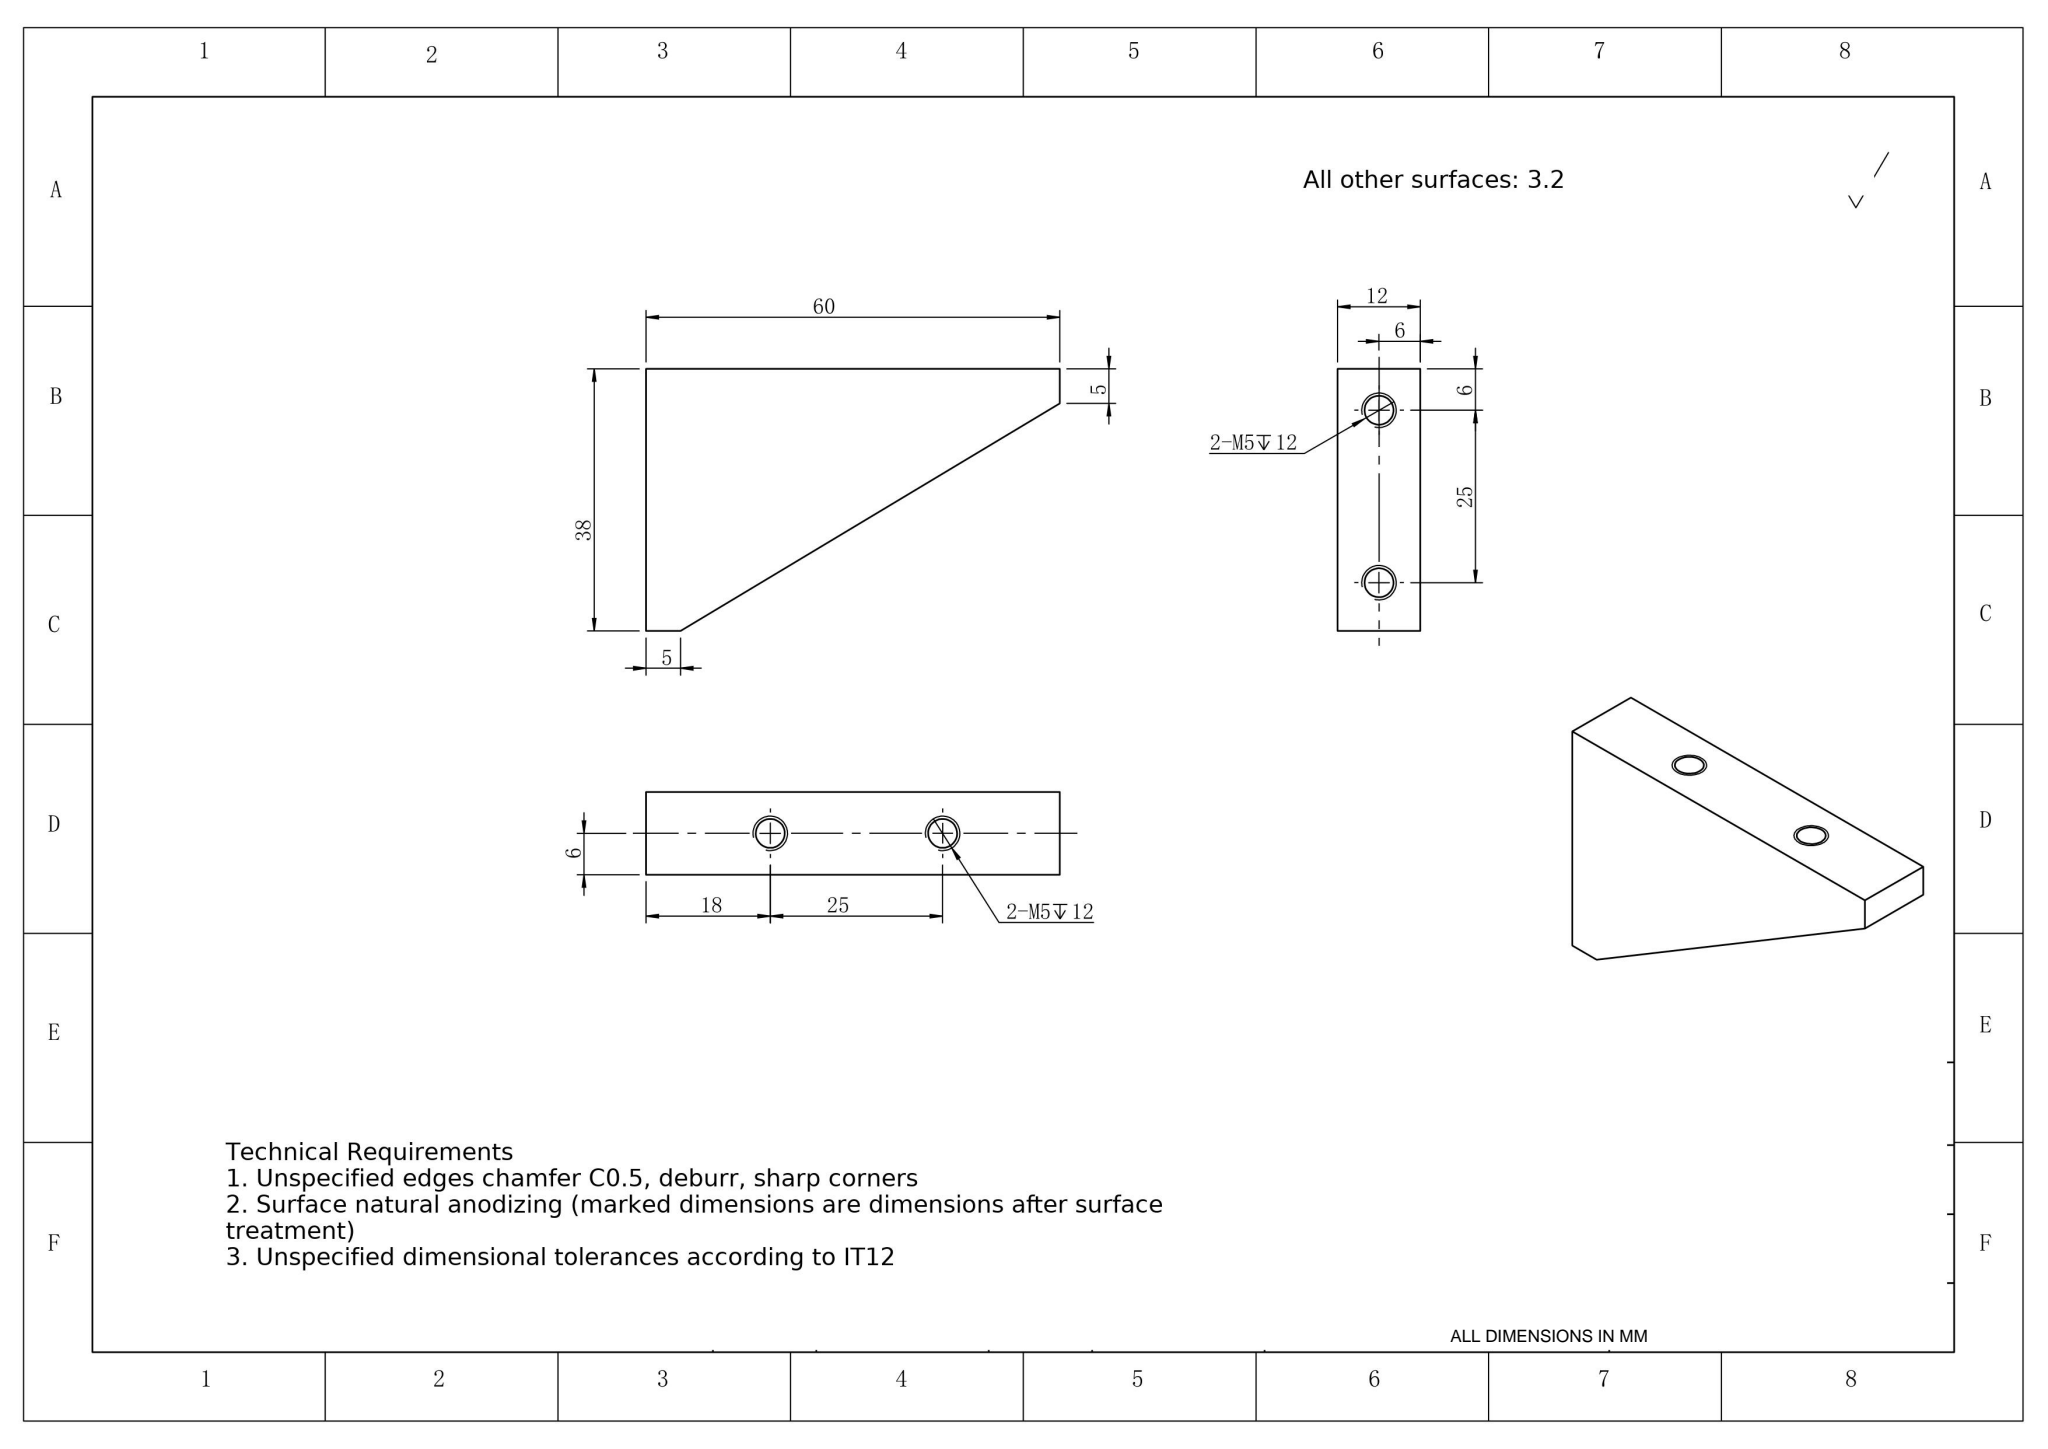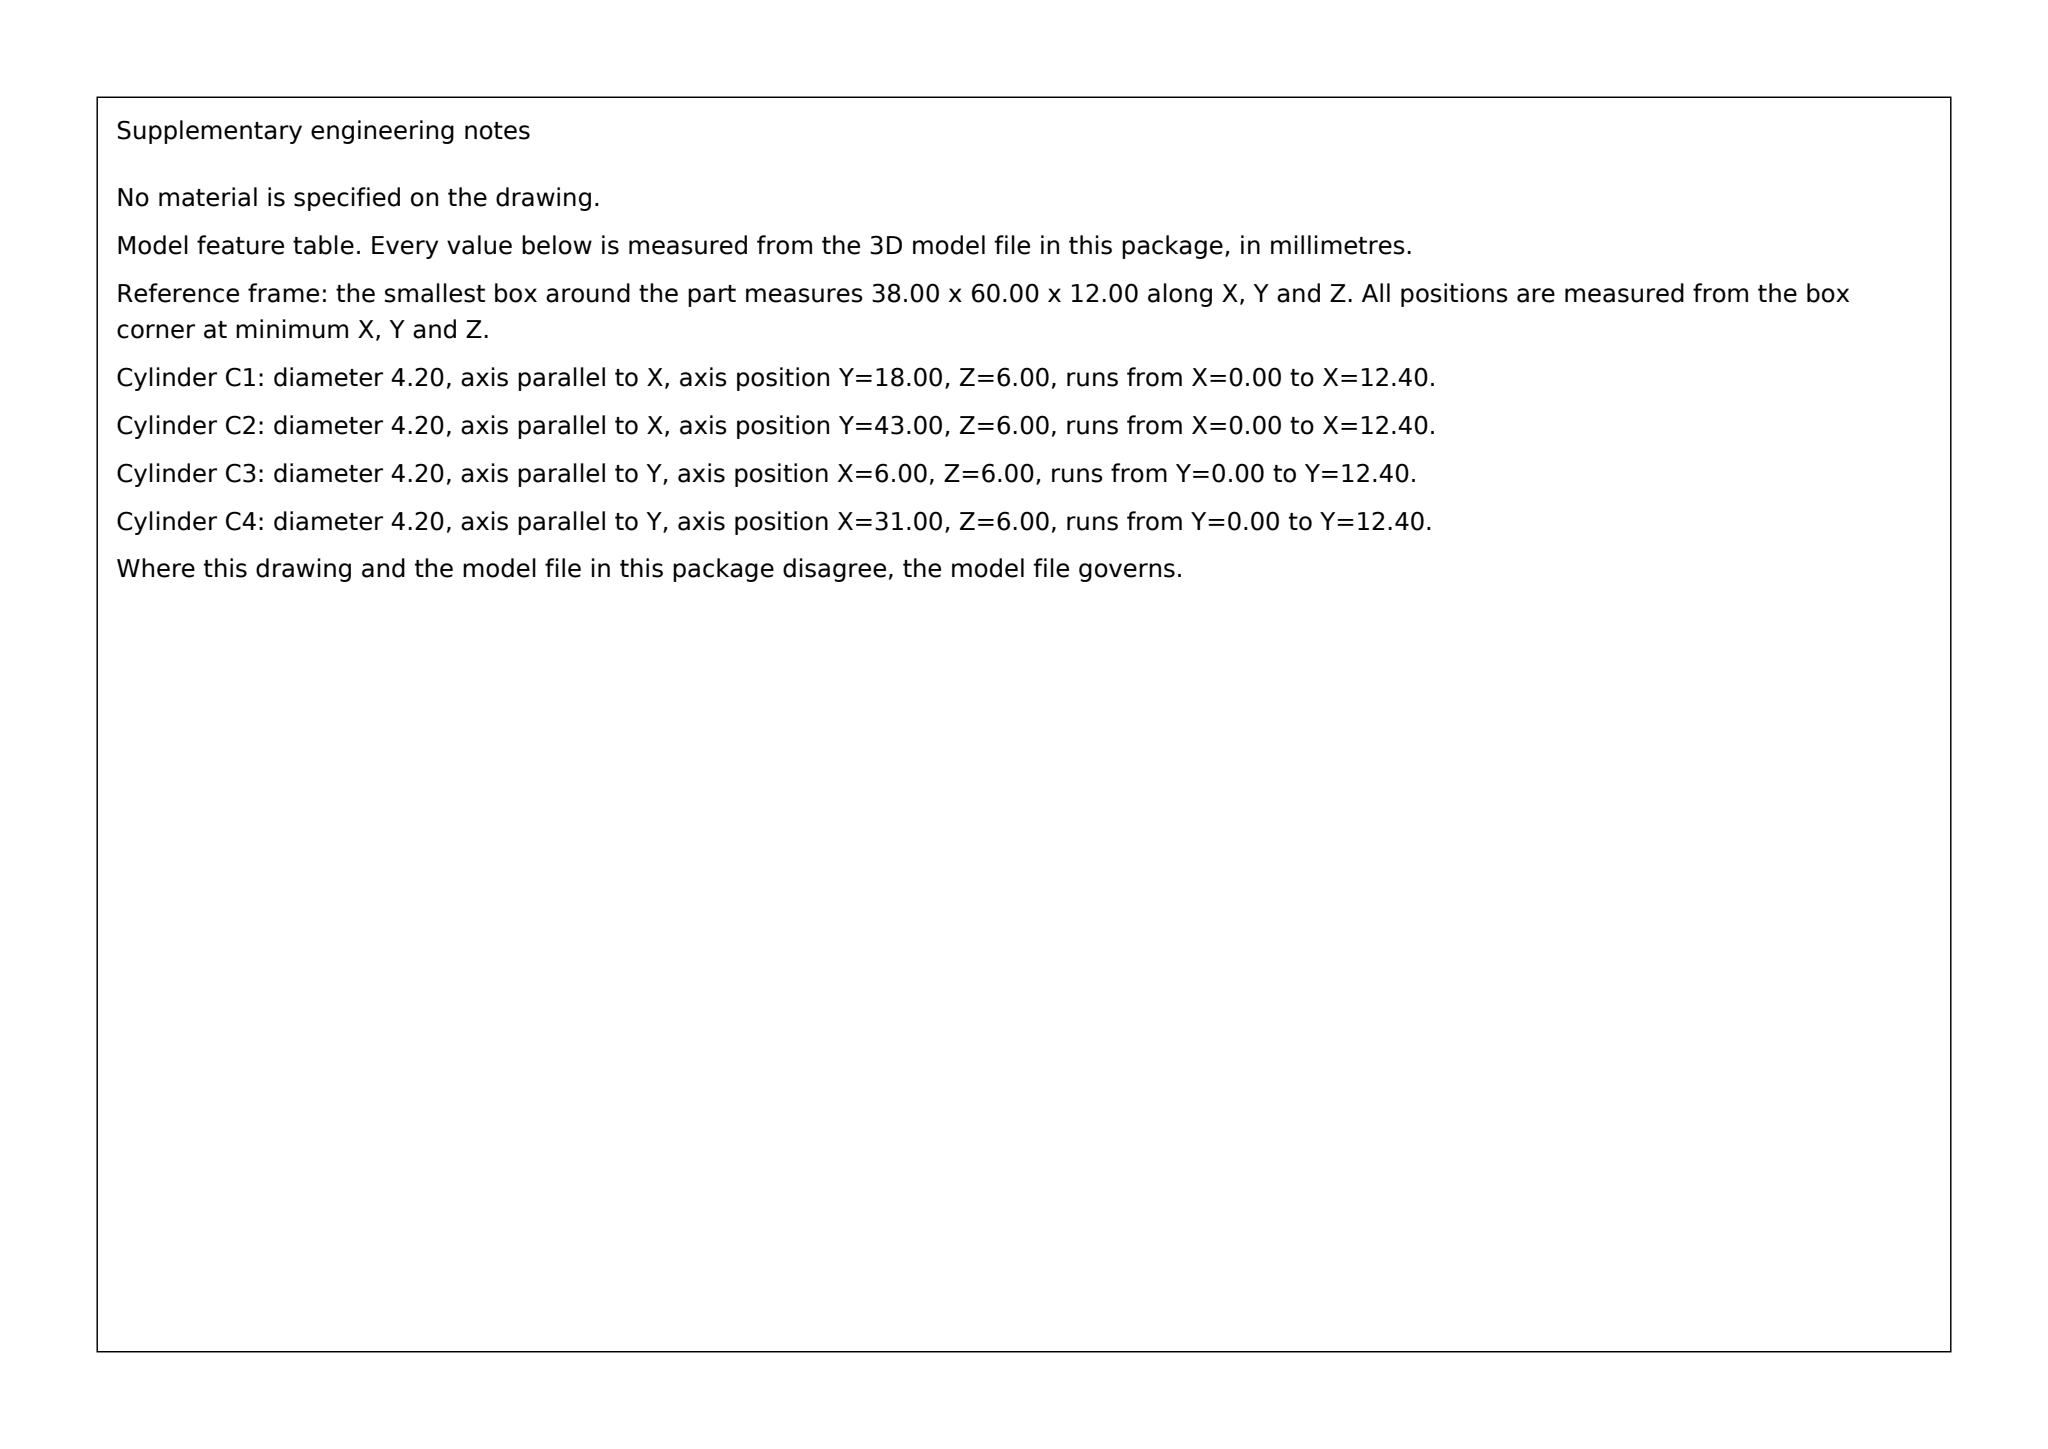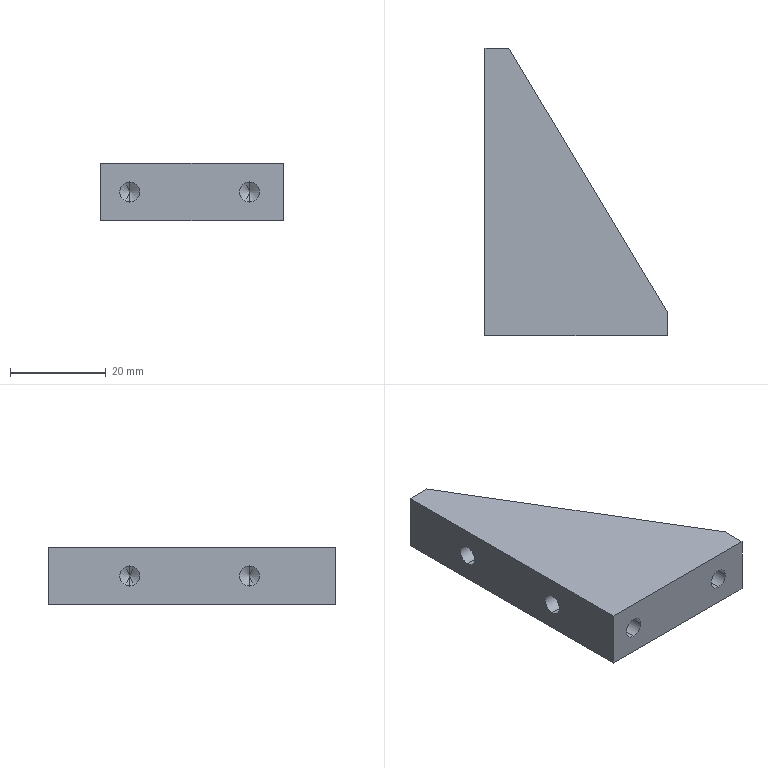Part | SolidWorks | mm | 1 solid | 23 faces | box 38 x 60 x 12 mm | volume 15760 mm3 | cylinder 8 | cone 8 | plane 7 | commonest cylinder face diameters 4.2 x8
build123d program:
from build123d import *

# Parameters (mm, degrees)
BOSS_EXTRUDE1_DEPTH   = 6
M5_TAPPED_HOLE1_D     = 4.2
M5_TAPPED_HOLE1_DEPTH = 12.4
M5_TAPPED_HOLE1_TIP   = 1.262
M5_TAPPED_HOLE2_D     = 4.2
M5_TAPPED_HOLE2_DEPTH = 12.4
M5_TAPPED_HOLE2_TIP   = 1.262


with BuildPart() as part:
    # Sketch1 → Boss-Extrude1 (new, symmetric)
    with BuildSketch(Plane.XY):
        Polygon((0, 60), (0, 0), (38, 0), (38, 5), (5, 60), align=None)
    extrude(amount=BOSS_EXTRUDE1_DEPTH, both=True)

    # M5 Tapped Hole1
    with Locations(Plane.ZY):
        with Locations((0, 18), (0, 43)):
            Hole(M5_TAPPED_HOLE1_D / 2, depth=M5_TAPPED_HOLE1_DEPTH)
            with Locations((0, 0, -(M5_TAPPED_HOLE1_DEPTH + M5_TAPPED_HOLE1_TIP / 2))):  # 118° drill point
                Cone(0, M5_TAPPED_HOLE1_D / 2, M5_TAPPED_HOLE1_TIP, mode=Mode.SUBTRACT)

    # M5 Tapped Hole2
    with Locations(Plane(origin=(0, 0, 0), x_dir=(-1, 0, 0), z_dir=(0, -1, 0))):
        with Locations((-31, 0), (-6, 0)):
            Hole(M5_TAPPED_HOLE2_D / 2, depth=M5_TAPPED_HOLE2_DEPTH)
            with Locations((0, 0, -(M5_TAPPED_HOLE2_DEPTH + M5_TAPPED_HOLE2_TIP / 2))):  # 118° drill point
                Cone(0, M5_TAPPED_HOLE2_D / 2, M5_TAPPED_HOLE2_TIP, mode=Mode.SUBTRACT)


solid = part.part